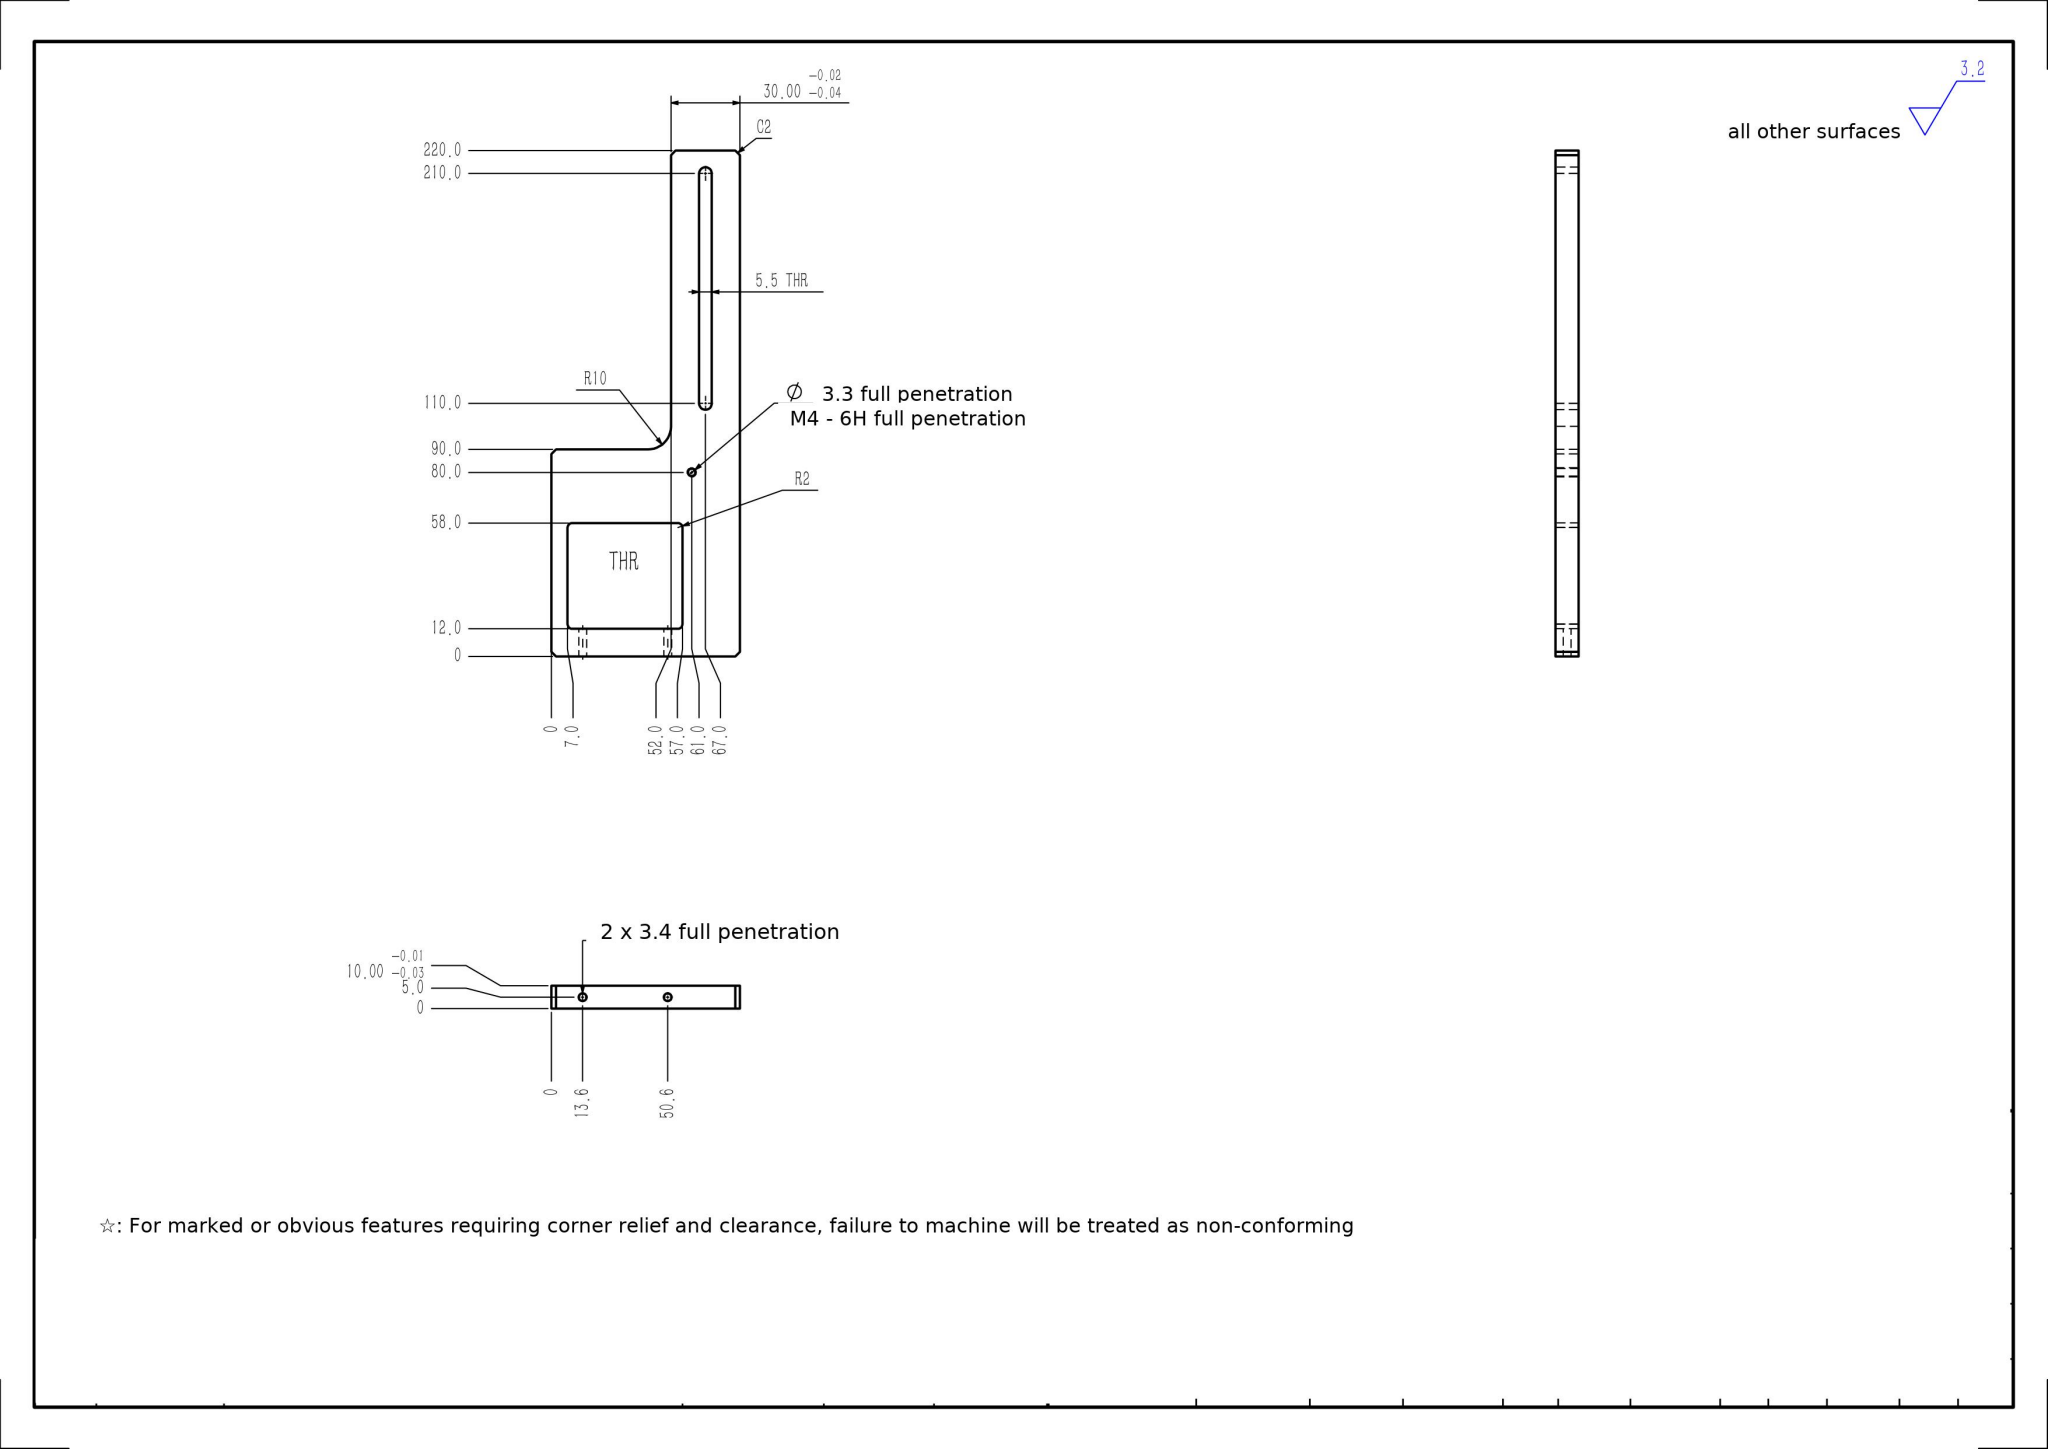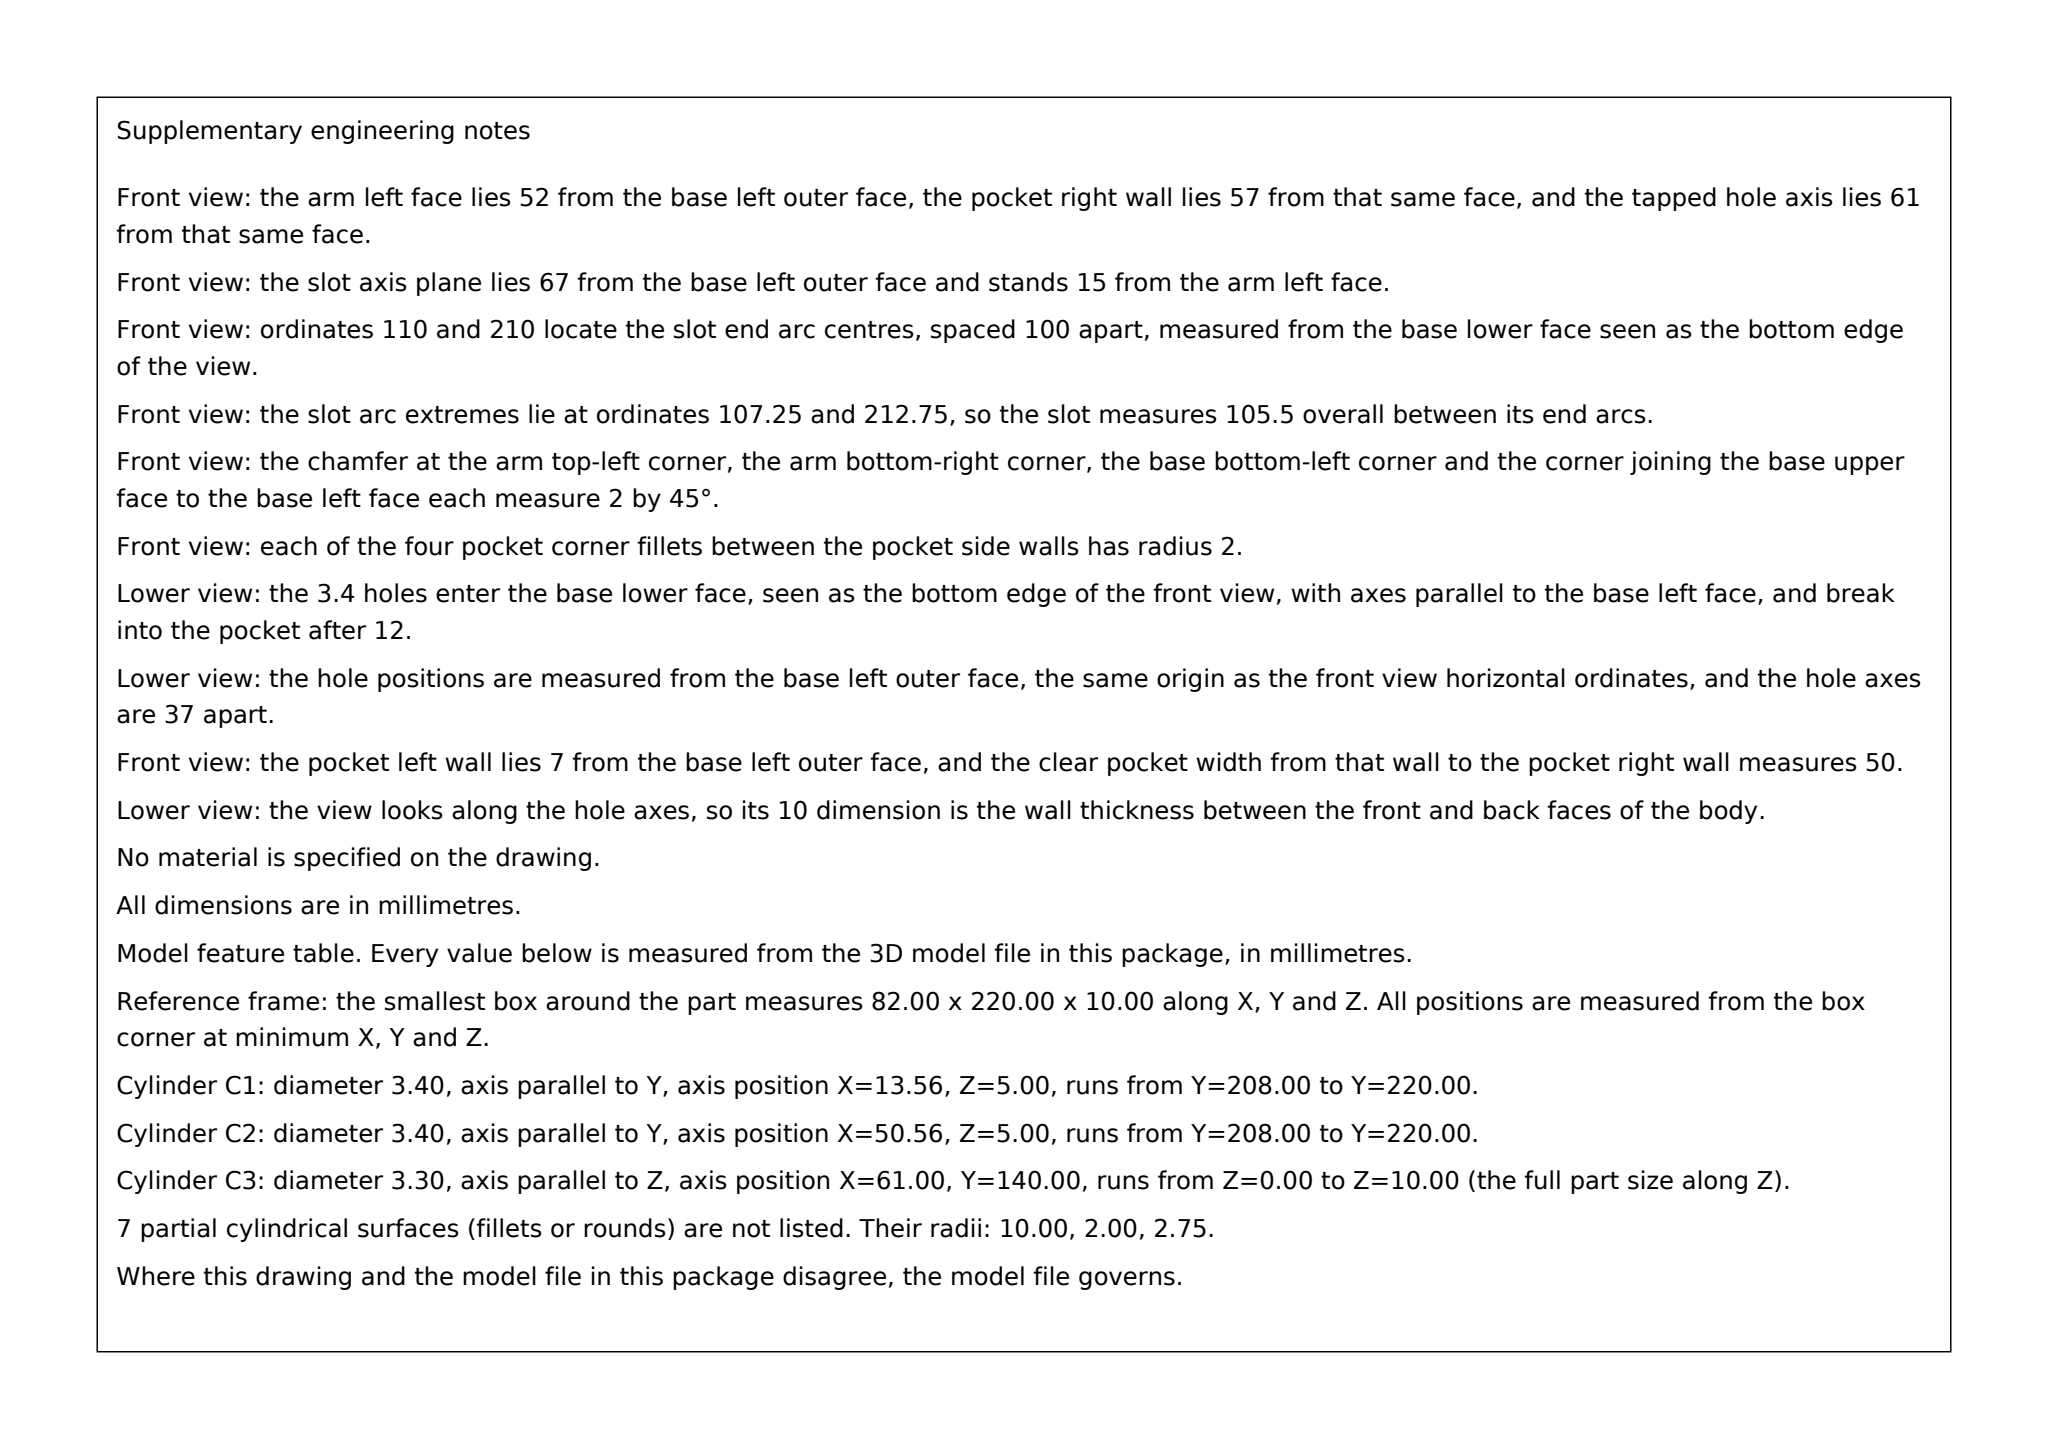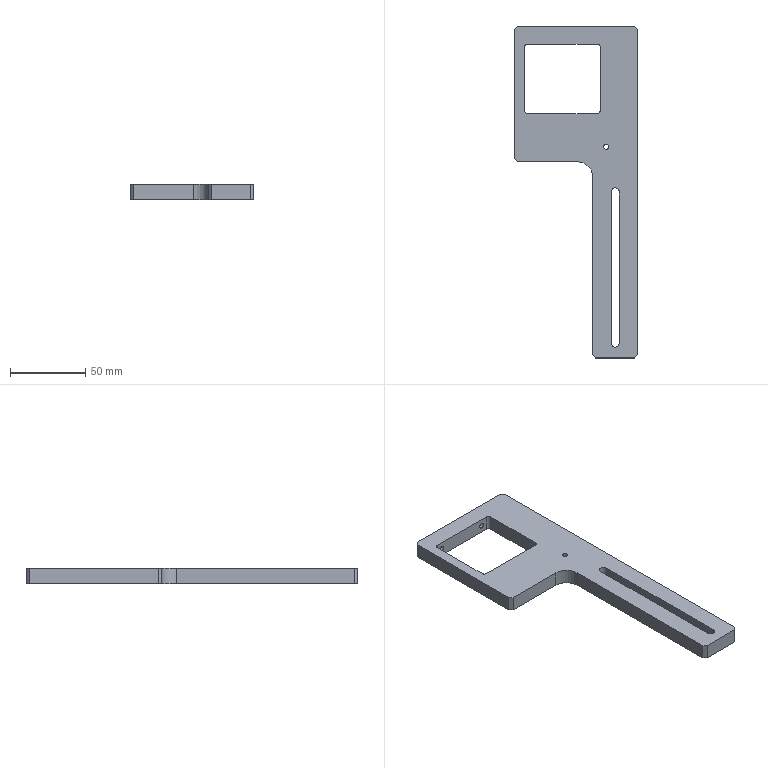Part | SolidWorks | mm | 1 solid | 32 faces | box 82 x 220 x 10 mm | volume 83908 mm3 | plane 19 | cylinder 13 | commonest cylinder face diameters 3.4 x4 4 x4 3.3 x2 5.5 x2 20 x1
Drawing notes:
Ø3.3 THRU, M4-6H THRU (10 THK PLATE) AT X61, Y80 | from the solid: cylinder dia 3.3, axis z, pos [61,140], length 10 = full plate thk (z planes 0 and 10)